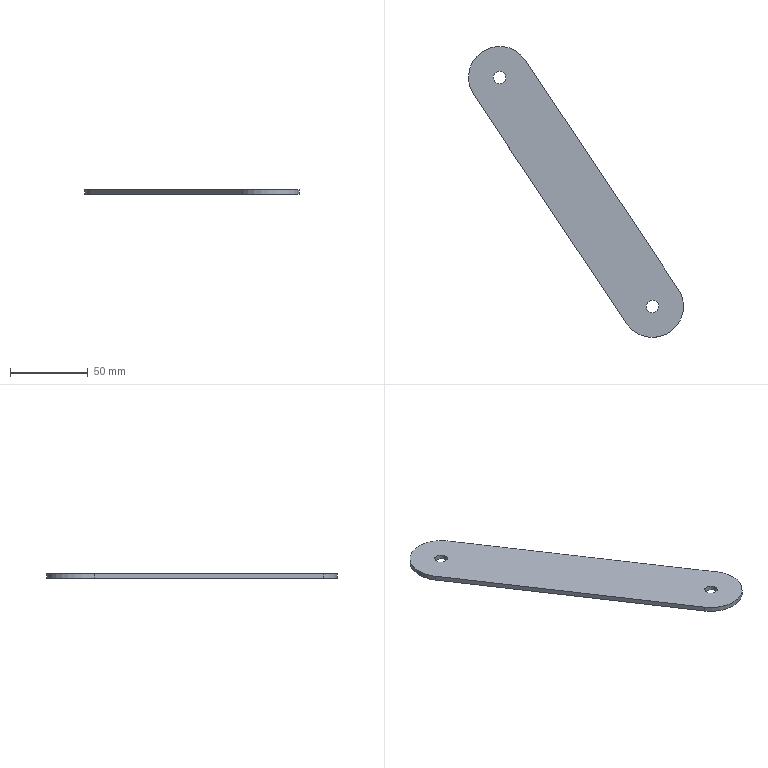Component | SolidWorks | 40 MM KOL-1 | 1 solid | 11 faces | box 138.33 x 187.17 x 3 mm | volume 24708 mm3 | cylinder 7 | plane 4 | commonest cylinder face diameters 8 x4 40 x3
STEP:
#1=CARTESIAN_POINT('',(5.226,6.635,-14.253));
#2=VERTEX_POINT('',#1);
#3=CARTESIAN_POINT('',(5.051,6.897,-14.253));
#4=VERTEX_POINT('',#3);
#5=CARTESIAN_POINT('',(5.139,6.766,-14.253));
#6=DIRECTION('',(0.,0.,1.));
#7=DIRECTION('',(-0.5556,0.8315,0.));
#8=AXIS2_PLACEMENT_3D('',#5,#6,#7);
#9=CIRCLE('',#8,0.1575);
#10=EDGE_CURVE('',#2,#4,#9,.T.);
#11=ORIENTED_EDGE('',*,*,#10,.F.);
#12=CARTESIAN_POINT('',(5.226,6.635,-14.135));
#13=VERTEX_POINT('',#12);
#14=CARTESIAN_POINT('',(5.226,6.635,-14.253));
#15=DIRECTION('',(0.,0.,1.));
#16=VECTOR('',#15,39.37);
#17=LINE('',#14,#16);
#18=EDGE_CURVE('',#2,#13,#17,.T.);
#19=ORIENTED_EDGE('',*,*,#18,.T.);
#20=CARTESIAN_POINT('',(5.051,6.897,-14.135));
#21=VERTEX_POINT('',#20);
#22=CARTESIAN_POINT('',(5.139,6.766,-14.135));
#23=DIRECTION('',(0.,0.,1.));
#24=DIRECTION('',(-0.5556,0.8315,0.));
#25=AXIS2_PLACEMENT_3D('',#22,#23,#24);
#26=CIRCLE('',#25,0.1575);
#27=EDGE_CURVE('',#13,#21,#26,.T.);
#28=ORIENTED_EDGE('',*,*,#27,.T.);
#29=CARTESIAN_POINT('',(5.051,6.897,-14.253));
#30=DIRECTION('',(0.,0.,1.));
#31=VECTOR('',#30,39.37);
#32=LINE('',#29,#31);
#33=EDGE_CURVE('',#4,#21,#32,.T.);
#34=ORIENTED_EDGE('',*,*,#33,.F.);
#35=EDGE_LOOP('',(#11,#19,#28,#34));
#36=FACE_OUTER_BOUND('',#35,.T.);
#37=CARTESIAN_POINT('',(5.139,6.766,-14.253));
#38=DIRECTION('',(0.,0.,1.));
#39=DIRECTION('',(-0.5556,0.8315,0.));
#40=AXIS2_PLACEMENT_3D('',#37,#38,#39);
#41=CYLINDRICAL_SURFACE('',#40,0.1575);
#42=ADVANCED_FACE('',(#36),#41,.F.);
#43=CARTESIAN_POINT('',(9.097,0.8406,-14.253));
#44=VERTEX_POINT('',#43);
#45=CARTESIAN_POINT('',(8.922,1.102,-14.253));
#46=VERTEX_POINT('',#45);
#47=CARTESIAN_POINT('',(9.01,0.9715,-14.253));
#48=DIRECTION('',(0.,0.,1.));
#49=DIRECTION('',(-0.5556,0.8315,0.));
#50=AXIS2_PLACEMENT_3D('',#47,#48,#49);
#51=CIRCLE('',#50,0.1575);
#52=EDGE_CURVE('',#44,#46,#51,.T.);
#53=ORIENTED_EDGE('',*,*,#52,.F.);
#54=CARTESIAN_POINT('',(9.097,0.8406,-14.135));
#55=VERTEX_POINT('',#54);
#56=CARTESIAN_POINT('',(9.097,0.8406,-14.253));
#57=DIRECTION('',(0.,0.,1.));
#58=VECTOR('',#57,39.37);
#59=LINE('',#56,#58);
#60=EDGE_CURVE('',#44,#55,#59,.T.);
#61=ORIENTED_EDGE('',*,*,#60,.T.);
#62=CARTESIAN_POINT('',(8.922,1.102,-14.135));
#63=VERTEX_POINT('',#62);
#64=CARTESIAN_POINT('',(9.01,0.9715,-14.135));
#65=DIRECTION('',(0.,0.,1.));
#66=DIRECTION('',(-0.5556,0.8315,0.));
#67=AXIS2_PLACEMENT_3D('',#64,#65,#66);
#68=CIRCLE('',#67,0.1575);
#69=EDGE_CURVE('',#55,#63,#68,.T.);
#70=ORIENTED_EDGE('',*,*,#69,.T.);
#71=CARTESIAN_POINT('',(8.922,1.102,-14.253));
#72=DIRECTION('',(0.,0.,1.));
#73=VECTOR('',#72,39.37);
#74=LINE('',#71,#73);
#75=EDGE_CURVE('',#46,#63,#74,.T.);
#76=ORIENTED_EDGE('',*,*,#75,.F.);
#77=EDGE_LOOP('',(#53,#61,#70,#76));
#78=FACE_OUTER_BOUND('',#77,.T.);
#79=CARTESIAN_POINT('',(9.01,0.9715,-14.253));
#80=DIRECTION('',(0.,0.,1.));
#81=DIRECTION('',(-0.5556,0.8315,0.));
#82=AXIS2_PLACEMENT_3D('',#79,#80,#81);
#83=CYLINDRICAL_SURFACE('',#82,0.1575);
#84=ADVANCED_FACE('',(#78),#83,.F.);
#85=CARTESIAN_POINT('',(5.793,7.203,-14.253));
#86=VERTEX_POINT('',#85);
#87=CARTESIAN_POINT('',(4.701,7.42,-14.253));
#88=VERTEX_POINT('',#87);
#89=CARTESIAN_POINT('',(5.139,6.766,-14.253));
#90=DIRECTION('',(0.,0.,1.));
#91=DIRECTION('',(-0.5556,0.8315,0.));
#92=AXIS2_PLACEMENT_3D('',#89,#90,#91);
#93=CIRCLE('',#92,0.7874);
#94=EDGE_CURVE('',#86,#88,#93,.T.);
#95=ORIENTED_EDGE('',*,*,#94,.T.);
#96=CARTESIAN_POINT('',(4.701,7.42,-14.135));
#97=VERTEX_POINT('',#96);
#98=CARTESIAN_POINT('',(4.701,7.42,-14.253));
#99=DIRECTION('',(0.,0.,1.));
#100=VECTOR('',#99,39.37);
#101=LINE('',#98,#100);
#102=EDGE_CURVE('',#88,#97,#101,.T.);
#103=ORIENTED_EDGE('',*,*,#102,.T.);
#104=CARTESIAN_POINT('',(5.793,7.203,-14.135));
#105=VERTEX_POINT('',#104);
#106=CARTESIAN_POINT('',(5.139,6.766,-14.135));
#107=DIRECTION('',(0.,0.,1.));
#108=DIRECTION('',(-0.5556,0.8315,0.));
#109=AXIS2_PLACEMENT_3D('',#106,#107,#108);
#110=CIRCLE('',#109,0.7874);
#111=EDGE_CURVE('',#105,#97,#110,.T.);
#112=ORIENTED_EDGE('',*,*,#111,.F.);
#113=CARTESIAN_POINT('',(5.793,7.203,-14.253));
#114=DIRECTION('',(0.,0.,1.));
#115=VECTOR('',#114,39.37);
#116=LINE('',#113,#115);
#117=EDGE_CURVE('',#86,#105,#116,.T.);
#118=ORIENTED_EDGE('',*,*,#117,.F.);
#119=EDGE_LOOP('',(#95,#103,#112,#118));
#120=FACE_OUTER_BOUND('',#119,.T.);
#121=CARTESIAN_POINT('',(5.139,6.766,-14.253));
#122=DIRECTION('',(0.,0.,1.));
#123=DIRECTION('',(-0.5556,0.8315,0.));
#124=AXIS2_PLACEMENT_3D('',#121,#122,#123);
#125=CYLINDRICAL_SURFACE('',#124,0.7874);
#126=ADVANCED_FACE('',(#120),#125,.T.);
#127=CARTESIAN_POINT('',(8.355,0.5341,-14.135));
#128=VERTEX_POINT('',#127);
#129=CARTESIAN_POINT('',(9.665,1.409,-14.135));
#130=VERTEX_POINT('',#129);
#131=CARTESIAN_POINT('',(9.01,0.9715,-14.135));
#132=DIRECTION('',(0.,0.,1.));
#133=DIRECTION('',(-0.5556,0.8315,0.));
#134=AXIS2_PLACEMENT_3D('',#131,#132,#133);
#135=CIRCLE('',#134,0.7874);
#136=EDGE_CURVE('',#128,#130,#135,.T.);
#137=ORIENTED_EDGE('',*,*,#136,.F.);
#138=CARTESIAN_POINT('',(8.355,0.5341,-14.253));
#139=VERTEX_POINT('',#138);
#140=CARTESIAN_POINT('',(8.355,0.5341,-14.253));
#141=DIRECTION('',(0.,0.,1.));
#142=VECTOR('',#141,39.37);
#143=LINE('',#140,#142);
#144=EDGE_CURVE('',#139,#128,#143,.T.);
#145=ORIENTED_EDGE('',*,*,#144,.F.);
#146=CARTESIAN_POINT('',(9.665,1.409,-14.253));
#147=VERTEX_POINT('',#146);
#148=CARTESIAN_POINT('',(9.01,0.9715,-14.253));
#149=DIRECTION('',(0.,0.,1.));
#150=DIRECTION('',(-0.5556,0.8315,0.));
#151=AXIS2_PLACEMENT_3D('',#148,#149,#150);
#152=CIRCLE('',#151,0.7874);
#153=EDGE_CURVE('',#139,#147,#152,.T.);
#154=ORIENTED_EDGE('',*,*,#153,.T.);
#155=CARTESIAN_POINT('',(9.665,1.409,-14.253));
#156=DIRECTION('',(0.,0.,1.));
#157=VECTOR('',#156,39.37);
#158=LINE('',#155,#157);
#159=EDGE_CURVE('',#147,#130,#158,.T.);
#160=ORIENTED_EDGE('',*,*,#159,.T.);
#161=EDGE_LOOP('',(#137,#145,#154,#160));
#162=FACE_OUTER_BOUND('',#161,.T.);
#163=CARTESIAN_POINT('',(9.01,0.9715,-14.253));
#164=DIRECTION('',(0.,0.,1.));
#165=DIRECTION('',(-0.5556,0.8315,0.));
#166=AXIS2_PLACEMENT_3D('',#163,#164,#165);
#167=CYLINDRICAL_SURFACE('',#166,0.7874);
#168=ADVANCED_FACE('',(#162),#167,.T.);
#169=CARTESIAN_POINT('',(4.484,6.328,-14.135));
#170=VERTEX_POINT('',#169);
#171=CARTESIAN_POINT('',(8.355,0.5341,-14.135));
#172=DIRECTION('',(0.5556,-0.8315,-0.));
#173=VECTOR('',#172,39.37);
#174=LINE('',#171,#173);
#175=EDGE_CURVE('',#170,#128,#174,.T.);
#176=ORIENTED_EDGE('',*,*,#175,.F.);
#177=CARTESIAN_POINT('',(4.484,6.328,-14.253));
#178=VERTEX_POINT('',#177);
#179=CARTESIAN_POINT('',(4.484,6.328,-14.253));
#180=DIRECTION('',(0.,0.,1.));
#181=VECTOR('',#180,39.37);
#182=LINE('',#179,#181);
#183=EDGE_CURVE('',#178,#170,#182,.T.);
#184=ORIENTED_EDGE('',*,*,#183,.F.);
#185=CARTESIAN_POINT('',(8.355,0.5341,-14.253));
#186=DIRECTION('',(0.5556,-0.8315,-0.));
#187=VECTOR('',#186,39.37);
#188=LINE('',#185,#187);
#189=EDGE_CURVE('',#178,#139,#188,.T.);
#190=ORIENTED_EDGE('',*,*,#189,.T.);
#191=ORIENTED_EDGE('',*,*,#144,.T.);
#192=EDGE_LOOP('',(#176,#184,#190,#191));
#193=FACE_OUTER_BOUND('',#192,.T.);
#194=CARTESIAN_POINT('',(8.355,0.5341,-14.253));
#195=DIRECTION('',(-0.8315,-0.5556,0.));
#196=DIRECTION('',(0.,0.,1.));
#197=AXIS2_PLACEMENT_3D('',#194,#195,#196);
#198=PLANE('',#197);
#199=ADVANCED_FACE('',(#193),#198,.T.);
#200=ORIENTED_EDGE('',*,*,#102,.F.);
#201=CARTESIAN_POINT('',(5.139,6.766,-14.253));
#202=DIRECTION('',(0.,0.,1.));
#203=DIRECTION('',(-0.5556,0.8315,0.));
#204=AXIS2_PLACEMENT_3D('',#201,#202,#203);
#205=CIRCLE('',#204,0.7874);
#206=EDGE_CURVE('',#88,#178,#205,.T.);
#207=ORIENTED_EDGE('',*,*,#206,.T.);
#208=ORIENTED_EDGE('',*,*,#183,.T.);
#209=CARTESIAN_POINT('',(5.139,6.766,-14.135));
#210=DIRECTION('',(0.,0.,1.));
#211=DIRECTION('',(-0.5556,0.8315,0.));
#212=AXIS2_PLACEMENT_3D('',#209,#210,#211);
#213=CIRCLE('',#212,0.7874);
#214=EDGE_CURVE('',#97,#170,#213,.T.);
#215=ORIENTED_EDGE('',*,*,#214,.F.);
#216=EDGE_LOOP('',(#200,#207,#208,#215));
#217=FACE_OUTER_BOUND('',#216,.T.);
#218=CARTESIAN_POINT('',(5.139,6.766,-14.253));
#219=DIRECTION('',(0.,0.,1.));
#220=DIRECTION('',(-0.5556,0.8315,0.));
#221=AXIS2_PLACEMENT_3D('',#218,#219,#220);
#222=CYLINDRICAL_SURFACE('',#221,0.7874);
#223=ADVANCED_FACE('',(#217),#222,.T.);
#224=CARTESIAN_POINT('',(9.665,1.409,-14.135));
#225=DIRECTION('',(-0.5556,0.8315,0.));
#226=VECTOR('',#225,39.37);
#227=LINE('',#224,#226);
#228=EDGE_CURVE('',#130,#105,#227,.T.);
#229=ORIENTED_EDGE('',*,*,#228,.F.);
#230=ORIENTED_EDGE('',*,*,#159,.F.);
#231=CARTESIAN_POINT('',(9.665,1.409,-14.253));
#232=DIRECTION('',(-0.5556,0.8315,0.));
#233=VECTOR('',#232,39.37);
#234=LINE('',#231,#233);
#235=EDGE_CURVE('',#147,#86,#234,.T.);
#236=ORIENTED_EDGE('',*,*,#235,.T.);
#237=ORIENTED_EDGE('',*,*,#117,.T.);
#238=EDGE_LOOP('',(#229,#230,#236,#237));
#239=FACE_OUTER_BOUND('',#238,.T.);
#240=CARTESIAN_POINT('',(9.665,1.409,-14.253));
#241=DIRECTION('',(0.8315,0.5556,-0.));
#242=DIRECTION('',(-0.,-0.,-1.));
#243=AXIS2_PLACEMENT_3D('',#240,#241,#242);
#244=PLANE('',#243);
#245=ADVANCED_FACE('',(#239),#244,.T.);
#246=CARTESIAN_POINT('',(5.139,6.766,-14.253));
#247=DIRECTION('',(0.,0.,1.));
#248=DIRECTION('',(-0.5556,0.8315,0.));
#249=AXIS2_PLACEMENT_3D('',#246,#247,#248);
#250=CIRCLE('',#249,0.1575);
#251=EDGE_CURVE('',#4,#2,#250,.T.);
#252=ORIENTED_EDGE('',*,*,#251,.T.);
#253=ORIENTED_EDGE('',*,*,#10,.T.);
#254=EDGE_LOOP('',(#252,#253));
#255=FACE_BOUND('',#254,.T.);
#256=CARTESIAN_POINT('',(9.01,0.9715,-14.253));
#257=DIRECTION('',(0.,0.,1.));
#258=DIRECTION('',(-0.5556,0.8315,0.));
#259=AXIS2_PLACEMENT_3D('',#256,#257,#258);
#260=CIRCLE('',#259,0.1575);
#261=EDGE_CURVE('',#46,#44,#260,.T.);
#262=ORIENTED_EDGE('',*,*,#261,.T.);
#263=ORIENTED_EDGE('',*,*,#52,.T.);
#264=EDGE_LOOP('',(#262,#263));
#265=FACE_BOUND('',#264,.T.);
#266=ORIENTED_EDGE('',*,*,#153,.F.);
#267=ORIENTED_EDGE('',*,*,#189,.F.);
#268=ORIENTED_EDGE('',*,*,#206,.F.);
#269=ORIENTED_EDGE('',*,*,#94,.F.);
#270=ORIENTED_EDGE('',*,*,#235,.F.);
#271=EDGE_LOOP('',(#266,#267,#268,#269,#270));
#272=FACE_OUTER_BOUND('',#271,.T.);
#273=CARTESIAN_POINT('',(9.01,0.9715,-14.253));
#274=DIRECTION('',(0.,0.,1.));
#275=DIRECTION('',(-0.5556,0.8315,0.));
#276=AXIS2_PLACEMENT_3D('',#273,#274,#275);
#277=PLANE('',#276);
#278=ADVANCED_FACE('',(#255,#265,#272),#277,.F.);
#279=CARTESIAN_POINT('',(5.139,6.766,-14.135));
#280=DIRECTION('',(0.,0.,1.));
#281=DIRECTION('',(-0.5556,0.8315,0.));
#282=AXIS2_PLACEMENT_3D('',#279,#280,#281);
#283=CIRCLE('',#282,0.1575);
#284=EDGE_CURVE('',#21,#13,#283,.T.);
#285=ORIENTED_EDGE('',*,*,#284,.F.);
#286=ORIENTED_EDGE('',*,*,#27,.F.);
#287=EDGE_LOOP('',(#285,#286));
#288=FACE_BOUND('',#287,.T.);
#289=CARTESIAN_POINT('',(9.01,0.9715,-14.135));
#290=DIRECTION('',(0.,0.,1.));
#291=DIRECTION('',(-0.5556,0.8315,0.));
#292=AXIS2_PLACEMENT_3D('',#289,#290,#291);
#293=CIRCLE('',#292,0.1575);
#294=EDGE_CURVE('',#63,#55,#293,.T.);
#295=ORIENTED_EDGE('',*,*,#294,.F.);
#296=ORIENTED_EDGE('',*,*,#69,.F.);
#297=EDGE_LOOP('',(#295,#296));
#298=FACE_BOUND('',#297,.T.);
#299=ORIENTED_EDGE('',*,*,#136,.T.);
#300=ORIENTED_EDGE('',*,*,#228,.T.);
#301=ORIENTED_EDGE('',*,*,#111,.T.);
#302=ORIENTED_EDGE('',*,*,#214,.T.);
#303=ORIENTED_EDGE('',*,*,#175,.T.);
#304=EDGE_LOOP('',(#299,#300,#301,#302,#303));
#305=FACE_OUTER_BOUND('',#304,.T.);
#306=CARTESIAN_POINT('',(9.01,0.9715,-14.135));
#307=DIRECTION('',(0.,0.,1.));
#308=DIRECTION('',(-0.5556,0.8315,0.));
#309=AXIS2_PLACEMENT_3D('',#306,#307,#308);
#310=PLANE('',#309);
#311=ADVANCED_FACE('',(#288,#298,#305),#310,.T.);
#312=ORIENTED_EDGE('',*,*,#60,.F.);
#313=ORIENTED_EDGE('',*,*,#261,.F.);
#314=ORIENTED_EDGE('',*,*,#75,.T.);
#315=ORIENTED_EDGE('',*,*,#294,.T.);
#316=EDGE_LOOP('',(#312,#313,#314,#315));
#317=FACE_OUTER_BOUND('',#316,.T.);
#318=CARTESIAN_POINT('',(9.01,0.9715,-14.253));
#319=DIRECTION('',(0.,0.,1.));
#320=DIRECTION('',(-0.5556,0.8315,0.));
#321=AXIS2_PLACEMENT_3D('',#318,#319,#320);
#322=CYLINDRICAL_SURFACE('',#321,0.1575);
#323=ADVANCED_FACE('',(#317),#322,.F.);
#324=ORIENTED_EDGE('',*,*,#18,.F.);
#325=ORIENTED_EDGE('',*,*,#251,.F.);
#326=ORIENTED_EDGE('',*,*,#33,.T.);
#327=ORIENTED_EDGE('',*,*,#284,.T.);
#328=EDGE_LOOP('',(#324,#325,#326,#327));
#329=FACE_OUTER_BOUND('',#328,.T.);
#330=CARTESIAN_POINT('',(5.139,6.766,-14.253));
#331=DIRECTION('',(0.,0.,1.));
#332=DIRECTION('',(-0.5556,0.8315,0.));
#333=AXIS2_PLACEMENT_3D('',#330,#331,#332);
#334=CYLINDRICAL_SURFACE('',#333,0.1575);
#335=ADVANCED_FACE('',(#329),#334,.F.);
#336=CLOSED_SHELL('',(#42,#84,#126,#168,#199,#223,#245,#278,#311,#323,#335));
#337=MANIFOLD_SOLID_BREP('',#336);
#338=CARTESIAN_POINT('',(0.,0.,0.));
#339=DIRECTION('',(0.,0.,1.));
#340=DIRECTION('',(1.,0.,0.));
#341=AXIS2_PLACEMENT_3D('',#338,#339,#340);
#342=(LENGTH_UNIT()NAMED_UNIT(*)SI_UNIT($,.METRE.));
#343=LENGTH_MEASURE_WITH_UNIT(LENGTH_MEASURE(0.0254),#342);
#344=DIMENSIONAL_EXPONENTS(1.,0.,0.,0.,0.,0.,0.);
#345=(CONVERSION_BASED_UNIT('',#343)LENGTH_UNIT()NAMED_UNIT(#344));
#346=UNCERTAINTY_MEASURE_WITH_UNIT(LENGTH_MEASURE(0.00001),#345,'','');
#347=(NAMED_UNIT(*)PLANE_ANGLE_UNIT()SI_UNIT($,.RADIAN.));
#348=(NAMED_UNIT(*)SI_UNIT($,.STERADIAN.)SOLID_ANGLE_UNIT());
#349=(GEOMETRIC_REPRESENTATION_CONTEXT(3)GLOBAL_UNCERTAINTY_ASSIGNED_CONTEXT((#346))GLOBAL_UNIT_ASSIGNED_CONTEXT((#345,#347,#348))REPRESENTATION_CONTEXT('',''));
#350=ADVANCED_BREP_SHAPE_REPRESENTATION('',(#337,#341),#349);
#351=COLOUR_RGB('',0.7922,0.8196,0.9333);
#352=FILL_AREA_STYLE_COLOUR('',#351);
#353=FILL_AREA_STYLE('',(#352));
#354=SURFACE_STYLE_FILL_AREA(#353);
#355=SURFACE_SIDE_STYLE('',(#354));
#356=SURFACE_STYLE_USAGE(.BOTH.,#355);
#357=PRESENTATION_STYLE_ASSIGNMENT((#356));
#358=STYLED_ITEM('',(#357),#337);
#359=PRESENTATION_LAYER_ASSIGNMENT('','',(#358));
#360=(LENGTH_UNIT()NAMED_UNIT(*)SI_UNIT($,.METRE.));
#361=LENGTH_MEASURE_WITH_UNIT(LENGTH_MEASURE(0.0254),#360);
#362=DIMENSIONAL_EXPONENTS(1.,0.,0.,0.,0.,0.,0.);
#363=(CONVERSION_BASED_UNIT('',#361)LENGTH_UNIT()NAMED_UNIT(#362));
#364=UNCERTAINTY_MEASURE_WITH_UNIT(LENGTH_MEASURE(0.00001),#363,'','');
#365=(NAMED_UNIT(*)PLANE_ANGLE_UNIT()SI_UNIT($,.RADIAN.));
#366=(NAMED_UNIT(*)SI_UNIT($,.STERADIAN.)SOLID_ANGLE_UNIT());
#367=(GEOMETRIC_REPRESENTATION_CONTEXT(3)GLOBAL_UNCERTAINTY_ASSIGNED_CONTEXT((#364))GLOBAL_UNIT_ASSIGNED_CONTEXT((#363,#365,#366))REPRESENTATION_CONTEXT('',''));
#368=MECHANICAL_DESIGN_GEOMETRIC_PRESENTATION_REPRESENTATION('',(#358),#367);